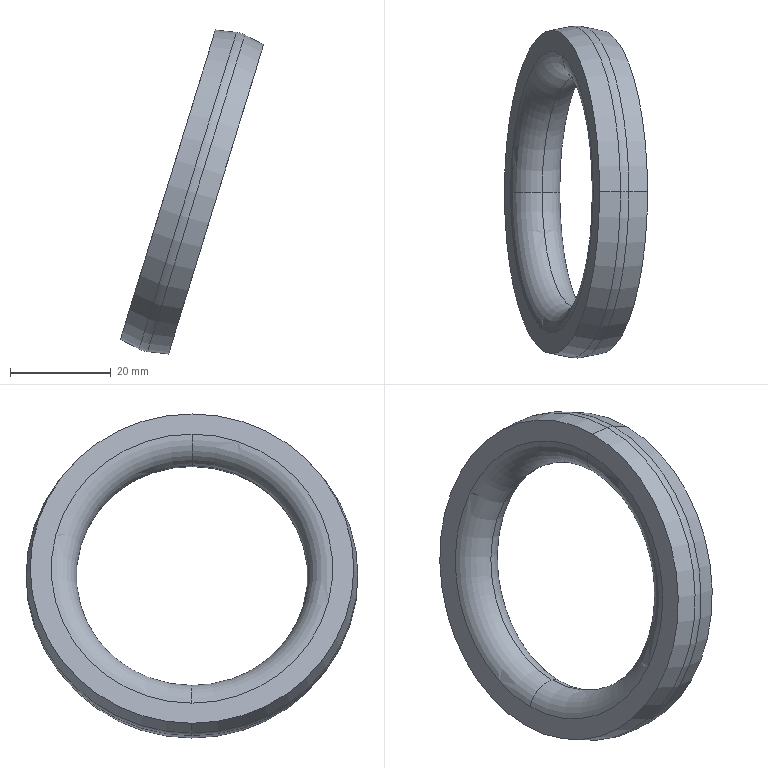Component | SolidWorks | DriveDevice-1_GuideWheelRubber-1 | 1 solid | 12 faces | box 28.47 x 66.09 x 64.5 mm | volume 15263 mm3 | torus 6 | cone 4 | plane 2
build123d program:
from build123d import *


with BuildPart() as part:
    # Sketch1 → Revolve1 (revolve)
    with BuildSketch(Plane(origin=(0, 0, 0), x_dir=(0, 0, -1), z_dir=(1, 0, 0)), mode=Mode.PRIVATE) as revolve1_sk:
        with BuildLine():
            Line((10, 28), (10, 32.2))
            Line((10, 32.2), (5.87, 32.964))
            ThreePointArc((5.87, 32.964), (5, 33.043), (4.13, 32.964))
            Line((4.13, 32.964), (0, 32.2))
            Line((0, 32.2), (0, 28))
            ThreePointArc((0, 28), (5, 23), (10, 28))
        make_face()
    revolve(revolve1_sk.sketch.rotate(Axis((0, 0, 5.5), (0, 0, -1)), 90), axis=Axis((0, 0, 5.5), (0, 0, -1)))


solid = part.part

# Placed as in the assembly
solid = solid.moved(Location((-210.893, 15, 15.882), (0, -72.922, -178.369)))
STEP:
#1=COLOUR_RGB('',0.7922,0.8196,0.9333);
#2=FILL_AREA_STYLE_COLOUR('',#1);
#3=FILL_AREA_STYLE('',(#2));
#4=SURFACE_STYLE_FILL_AREA(#3);
#5=SURFACE_SIDE_STYLE('',(#4));
#6=SURFACE_STYLE_USAGE(.BOTH.,#5);
#7=PRESENTATION_STYLE_ASSIGNMENT((#6));
#8=CARTESIAN_POINT('',(-8.381,0.5906,-0.2981));
#9=VERTEX_POINT('',#8);
#10=CARTESIAN_POINT('',(-8.25,0.5906,-0.5441));
#11=VERTEX_POINT('',#10);
#12=CARTESIAN_POINT('',(-8.438,0.5906,-0.4863));
#13=DIRECTION('',(-0.,1.,0.));
#14=DIRECTION('',(0.,-0.,1.));
#15=AXIS2_PLACEMENT_3D('',#12,#13,#14);
#16=CIRCLE('',#15,0.1969);
#17=EDGE_CURVE('',#9,#11,#16,.T.);
#18=ORIENTED_EDGE('',*,*,#17,.F.);
#19=CARTESIAN_POINT('',(-7.849,0.5906,1.433));
#20=VERTEX_POINT('',#19);
#21=CARTESIAN_POINT('',(-8.115,0.5906,0.5675));
#22=DIRECTION('',(-0.9559,-0.,0.2937));
#23=DIRECTION('',(0.2937,0.,0.9559));
#24=AXIS2_PLACEMENT_3D('',#21,#22,#23);
#25=CIRCLE('',#24,0.9055);
#26=EDGE_CURVE('',#9,#20,#25,.T.);
#27=ORIENTED_EDGE('',*,*,#26,.T.);
#28=CARTESIAN_POINT('',(-7.603,0.5906,1.563));
#29=VERTEX_POINT('',#28);
#30=CARTESIAN_POINT('',(-7.791,0.5906,1.621));
#31=DIRECTION('',(0.,-1.,-0.));
#32=DIRECTION('',(0.,0.,-1.));
#33=AXIS2_PLACEMENT_3D('',#30,#31,#32);
#34=CIRCLE('',#33,0.1969);
#35=EDGE_CURVE('',#20,#29,#34,.T.);
#36=ORIENTED_EDGE('',*,*,#35,.T.);
#37=CARTESIAN_POINT('',(-7.927,0.5906,0.5097));
#38=DIRECTION('',(-0.9559,-0.,0.2937));
#39=DIRECTION('',(0.2937,-0.,0.9559));
#40=AXIS2_PLACEMENT_3D('',#37,#38,#39);
#41=CIRCLE('',#40,1.102);
#42=EDGE_CURVE('',#11,#29,#41,.T.);
#43=ORIENTED_EDGE('',*,*,#42,.F.);
#44=EDGE_LOOP('',(#18,#27,#36,#43));
#45=FACE_OUTER_BOUND('',#44,.T.);
#46=CARTESIAN_POINT('',(-8.115,0.5906,0.5675));
#47=DIRECTION('',(-0.9559,-0.,0.2937));
#48=DIRECTION('',(0.2937,-0.,0.9559));
#49=AXIS2_PLACEMENT_3D('',#46,#47,#48);
#50=TOROIDAL_SURFACE('',#49,1.102,0.1969);
#51=ADVANCED_FACE('',(#45),#50,.T.);
#52=ORIENTED_EDGE('',*,*,#35,.F.);
#53=CARTESIAN_POINT('',(-8.115,0.5906,0.5675));
#54=DIRECTION('',(-0.9559,-0.,0.2937));
#55=DIRECTION('',(0.2937,0.,0.9559));
#56=AXIS2_PLACEMENT_3D('',#53,#54,#55);
#57=CIRCLE('',#56,0.9055);
#58=EDGE_CURVE('',#20,#9,#57,.T.);
#59=ORIENTED_EDGE('',*,*,#58,.T.);
#60=ORIENTED_EDGE('',*,*,#17,.T.);
#61=CARTESIAN_POINT('',(-7.927,0.5906,0.5097));
#62=DIRECTION('',(-0.9559,-0.,0.2937));
#63=DIRECTION('',(0.2937,-0.,0.9559));
#64=AXIS2_PLACEMENT_3D('',#61,#62,#63);
#65=CIRCLE('',#64,1.102);
#66=EDGE_CURVE('',#29,#11,#65,.T.);
#67=ORIENTED_EDGE('',*,*,#66,.F.);
#68=EDGE_LOOP('',(#52,#59,#60,#67));
#69=FACE_OUTER_BOUND('',#68,.T.);
#70=CARTESIAN_POINT('',(-8.115,0.5906,0.5675));
#71=DIRECTION('',(-0.9559,-0.,0.2937));
#72=DIRECTION('',(0.2937,-0.,0.9559));
#73=AXIS2_PLACEMENT_3D('',#70,#71,#72);
#74=TOROIDAL_SURFACE('',#73,1.102,0.1969);
#75=ADVANCED_FACE('',(#69),#74,.T.);
#76=CARTESIAN_POINT('',(-7.931,0.5906,1.837));
#77=VERTEX_POINT('',#76);
#78=CARTESIAN_POINT('',(-8.675,0.5906,-0.5865));
#79=VERTEX_POINT('',#78);
#80=CARTESIAN_POINT('',(-8.303,0.5906,0.6253));
#81=DIRECTION('',(-0.9559,-0.,0.2937));
#82=DIRECTION('',(0.2937,-0.,0.9559));
#83=AXIS2_PLACEMENT_3D('',#80,#81,#82);
#84=CIRCLE('',#83,1.268);
#85=EDGE_CURVE('',#77,#79,#84,.T.);
#86=ORIENTED_EDGE('',*,*,#85,.F.);
#87=CARTESIAN_POINT('',(-7.766,0.5906,1.818));
#88=VERTEX_POINT('',#87);
#89=CARTESIAN_POINT('',(-7.766,0.5906,1.818));
#90=DIRECTION('',(0.9934,0.,-0.115));
#91=VECTOR('',#90,39.37);
#92=LINE('',#89,#91);
#93=EDGE_CURVE('',#77,#88,#92,.T.);
#94=ORIENTED_EDGE('',*,*,#93,.T.);
#95=CARTESIAN_POINT('',(-8.529,0.5906,-0.663));
#96=VERTEX_POINT('',#95);
#97=CARTESIAN_POINT('',(-8.147,0.5906,0.5775));
#98=DIRECTION('',(-0.9559,-0.,0.2937));
#99=DIRECTION('',(0.2937,-0.,0.9559));
#100=AXIS2_PLACEMENT_3D('',#97,#98,#99);
#101=CIRCLE('',#100,1.298);
#102=EDGE_CURVE('',#88,#96,#101,.T.);
#103=ORIENTED_EDGE('',*,*,#102,.T.);
#104=CARTESIAN_POINT('',(-8.529,0.5906,-0.663));
#105=DIRECTION('',(0.8866,0.,-0.4626));
#106=VECTOR('',#105,39.37);
#107=LINE('',#104,#106);
#108=EDGE_CURVE('',#79,#96,#107,.T.);
#109=ORIENTED_EDGE('',*,*,#108,.F.);
#110=EDGE_LOOP('',(#86,#94,#103,#109));
#111=FACE_OUTER_BOUND('',#110,.T.);
#112=CARTESIAN_POINT('',(-8.147,0.5906,0.5775));
#113=DIRECTION('',(0.9559,0.,-0.2937));
#114=DIRECTION('',(-0.2937,0.,-0.9559));
#115=AXIS2_PLACEMENT_3D('',#112,#113,#114);
#116=CONICAL_SURFACE('',#115,1.298,0.1828);
#117=ADVANCED_FACE('',(#111),#116,.T.);
#118=CARTESIAN_POINT('',(-7.701,0.5906,1.798));
#119=VERTEX_POINT('',#118);
#120=CARTESIAN_POINT('',(-8.463,0.5906,-0.6831));
#121=VERTEX_POINT('',#120);
#122=CARTESIAN_POINT('',(-8.082,0.5906,0.5574));
#123=DIRECTION('',(-0.9559,-0.,0.2937));
#124=DIRECTION('',(0.2937,-0.,0.9559));
#125=AXIS2_PLACEMENT_3D('',#122,#123,#124);
#126=CIRCLE('',#125,1.298);
#127=EDGE_CURVE('',#119,#121,#126,.T.);
#128=ORIENTED_EDGE('',*,*,#127,.T.);
#129=CARTESIAN_POINT('',(-8.441,0.5906,-0.496));
#130=DIRECTION('',(-0.,1.,0.));
#131=DIRECTION('',(0.,-0.,1.));
#132=AXIS2_PLACEMENT_3D('',#129,#130,#131);
#133=CIRCLE('',#132,0.1884);
#134=EDGE_CURVE('',#121,#96,#133,.T.);
#135=ORIENTED_EDGE('',*,*,#134,.T.);
#136=ORIENTED_EDGE('',*,*,#102,.F.);
#137=CARTESIAN_POINT('',(-7.788,0.5906,1.631));
#138=DIRECTION('',(0.,-1.,-0.));
#139=DIRECTION('',(0.,0.,-1.));
#140=AXIS2_PLACEMENT_3D('',#137,#138,#139);
#141=CIRCLE('',#140,0.1884);
#142=EDGE_CURVE('',#119,#88,#141,.T.);
#143=ORIENTED_EDGE('',*,*,#142,.F.);
#144=EDGE_LOOP('',(#128,#135,#136,#143));
#145=FACE_OUTER_BOUND('',#144,.T.);
#146=CARTESIAN_POINT('',(-8.115,0.5906,0.5675));
#147=DIRECTION('',(-0.9559,-0.,0.2937));
#148=DIRECTION('',(0.2937,-0.,0.9559));
#149=AXIS2_PLACEMENT_3D('',#146,#147,#148);
#150=TOROIDAL_SURFACE('',#149,1.113,0.1884);
#151=ADVANCED_FACE('',(#145),#150,.T.);
#152=CARTESIAN_POINT('',(-7.554,0.5906,1.721));
#153=VERTEX_POINT('',#152);
#154=CARTESIAN_POINT('',(-8.299,0.5906,-0.7022));
#155=VERTEX_POINT('',#154);
#156=CARTESIAN_POINT('',(-7.927,0.5906,0.5097));
#157=DIRECTION('',(-0.9559,-0.,0.2937));
#158=DIRECTION('',(0.2937,-0.,0.9559));
#159=AXIS2_PLACEMENT_3D('',#156,#157,#158);
#160=CIRCLE('',#159,1.268);
#161=EDGE_CURVE('',#153,#155,#160,.T.);
#162=ORIENTED_EDGE('',*,*,#161,.T.);
#163=CARTESIAN_POINT('',(-8.299,0.5906,-0.7022));
#164=DIRECTION('',(-0.9934,-0.,0.115));
#165=VECTOR('',#164,39.37);
#166=LINE('',#163,#165);
#167=EDGE_CURVE('',#155,#121,#166,.T.);
#168=ORIENTED_EDGE('',*,*,#167,.T.);
#169=ORIENTED_EDGE('',*,*,#127,.F.);
#170=CARTESIAN_POINT('',(-7.554,0.5906,1.721));
#171=DIRECTION('',(-0.8866,-0.,0.4626));
#172=VECTOR('',#171,39.37);
#173=LINE('',#170,#172);
#174=EDGE_CURVE('',#153,#119,#173,.T.);
#175=ORIENTED_EDGE('',*,*,#174,.F.);
#176=EDGE_LOOP('',(#162,#168,#169,#175));
#177=FACE_OUTER_BOUND('',#176,.T.);
#178=CARTESIAN_POINT('',(-7.927,0.5906,0.5097));
#179=DIRECTION('',(-0.9559,-0.,0.2937));
#180=DIRECTION('',(0.2937,-0.,0.9559));
#181=AXIS2_PLACEMENT_3D('',#178,#179,#180);
#182=CONICAL_SURFACE('',#181,1.268,0.1828);
#183=ADVANCED_FACE('',(#177),#182,.T.);
#184=ORIENTED_EDGE('',*,*,#58,.F.);
#185=CARTESIAN_POINT('',(-7.979,0.5906,1.679));
#186=VERTEX_POINT('',#185);
#187=CARTESIAN_POINT('',(-7.791,0.5906,1.621));
#188=DIRECTION('',(0.,-1.,-0.));
#189=DIRECTION('',(0.,0.,-1.));
#190=AXIS2_PLACEMENT_3D('',#187,#188,#189);
#191=CIRCLE('',#190,0.1969);
#192=EDGE_CURVE('',#186,#20,#191,.T.);
#193=ORIENTED_EDGE('',*,*,#192,.F.);
#194=CARTESIAN_POINT('',(-8.627,0.5906,-0.4285));
#195=VERTEX_POINT('',#194);
#196=CARTESIAN_POINT('',(-8.303,0.5906,0.6253));
#197=DIRECTION('',(-0.9559,-0.,0.2937));
#198=DIRECTION('',(0.2937,-0.,0.9559));
#199=AXIS2_PLACEMENT_3D('',#196,#197,#198);
#200=CIRCLE('',#199,1.102);
#201=EDGE_CURVE('',#186,#195,#200,.T.);
#202=ORIENTED_EDGE('',*,*,#201,.T.);
#203=CARTESIAN_POINT('',(-8.438,0.5906,-0.4863));
#204=DIRECTION('',(-0.,1.,0.));
#205=DIRECTION('',(0.,-0.,1.));
#206=AXIS2_PLACEMENT_3D('',#203,#204,#205);
#207=CIRCLE('',#206,0.1969);
#208=EDGE_CURVE('',#195,#9,#207,.T.);
#209=ORIENTED_EDGE('',*,*,#208,.T.);
#210=EDGE_LOOP('',(#184,#193,#202,#209));
#211=FACE_OUTER_BOUND('',#210,.T.);
#212=CARTESIAN_POINT('',(-8.115,0.5906,0.5675));
#213=DIRECTION('',(-0.9559,-0.,0.2937));
#214=DIRECTION('',(0.2937,-0.,0.9559));
#215=AXIS2_PLACEMENT_3D('',#212,#213,#214);
#216=TOROIDAL_SURFACE('',#215,1.102,0.1969);
#217=ADVANCED_FACE('',(#211),#216,.T.);
#218=ORIENTED_EDGE('',*,*,#26,.F.);
#219=ORIENTED_EDGE('',*,*,#208,.F.);
#220=CARTESIAN_POINT('',(-8.303,0.5906,0.6253));
#221=DIRECTION('',(-0.9559,-0.,0.2937));
#222=DIRECTION('',(0.2937,-0.,0.9559));
#223=AXIS2_PLACEMENT_3D('',#220,#221,#222);
#224=CIRCLE('',#223,1.102);
#225=EDGE_CURVE('',#195,#186,#224,.T.);
#226=ORIENTED_EDGE('',*,*,#225,.T.);
#227=ORIENTED_EDGE('',*,*,#192,.T.);
#228=EDGE_LOOP('',(#218,#219,#226,#227));
#229=FACE_OUTER_BOUND('',#228,.T.);
#230=CARTESIAN_POINT('',(-8.115,0.5906,0.5675));
#231=DIRECTION('',(-0.9559,-0.,0.2937));
#232=DIRECTION('',(0.2937,-0.,0.9559));
#233=AXIS2_PLACEMENT_3D('',#230,#231,#232);
#234=TOROIDAL_SURFACE('',#233,1.102,0.1969);
#235=ADVANCED_FACE('',(#229),#234,.T.);
#236=ORIENTED_EDGE('',*,*,#161,.F.);
#237=CARTESIAN_POINT('',(-7.927,0.5906,0.5097));
#238=DIRECTION('',(-0.9559,-0.,0.2937));
#239=DIRECTION('',(0.2937,-0.,0.9559));
#240=AXIS2_PLACEMENT_3D('',#237,#238,#239);
#241=CIRCLE('',#240,1.268);
#242=EDGE_CURVE('',#155,#153,#241,.T.);
#243=ORIENTED_EDGE('',*,*,#242,.F.);
#244=EDGE_LOOP('',(#236,#243));
#245=FACE_OUTER_BOUND('',#244,.T.);
#246=ORIENTED_EDGE('',*,*,#66,.T.);
#247=ORIENTED_EDGE('',*,*,#42,.T.);
#248=EDGE_LOOP('',(#246,#247));
#249=FACE_BOUND('',#248,.T.);
#250=CARTESIAN_POINT('',(-7.927,1.693,0.5097));
#251=DIRECTION('',(-0.9559,-0.,0.2937));
#252=DIRECTION('',(0.2937,-0.,0.9559));
#253=AXIS2_PLACEMENT_3D('',#250,#251,#252);
#254=PLANE('',#253);
#255=ADVANCED_FACE('',(#245,#249),#254,.F.);
#256=ORIENTED_EDGE('',*,*,#167,.F.);
#257=ORIENTED_EDGE('',*,*,#242,.T.);
#258=ORIENTED_EDGE('',*,*,#174,.T.);
#259=CARTESIAN_POINT('',(-8.082,0.5906,0.5574));
#260=DIRECTION('',(-0.9559,-0.,0.2937));
#261=DIRECTION('',(0.2937,-0.,0.9559));
#262=AXIS2_PLACEMENT_3D('',#259,#260,#261);
#263=CIRCLE('',#262,1.298);
#264=EDGE_CURVE('',#121,#119,#263,.T.);
#265=ORIENTED_EDGE('',*,*,#264,.F.);
#266=EDGE_LOOP('',(#256,#257,#258,#265));
#267=FACE_OUTER_BOUND('',#266,.T.);
#268=CARTESIAN_POINT('',(-7.927,0.5906,0.5097));
#269=DIRECTION('',(-0.9559,-0.,0.2937));
#270=DIRECTION('',(0.2937,-0.,0.9559));
#271=AXIS2_PLACEMENT_3D('',#268,#269,#270);
#272=CONICAL_SURFACE('',#271,1.268,0.1828);
#273=ADVANCED_FACE('',(#267),#272,.T.);
#274=ORIENTED_EDGE('',*,*,#134,.F.);
#275=ORIENTED_EDGE('',*,*,#264,.T.);
#276=ORIENTED_EDGE('',*,*,#142,.T.);
#277=CARTESIAN_POINT('',(-8.147,0.5906,0.5775));
#278=DIRECTION('',(-0.9559,-0.,0.2937));
#279=DIRECTION('',(0.2937,-0.,0.9559));
#280=AXIS2_PLACEMENT_3D('',#277,#278,#279);
#281=CIRCLE('',#280,1.298);
#282=EDGE_CURVE('',#96,#88,#281,.T.);
#283=ORIENTED_EDGE('',*,*,#282,.F.);
#284=EDGE_LOOP('',(#274,#275,#276,#283));
#285=FACE_OUTER_BOUND('',#284,.T.);
#286=CARTESIAN_POINT('',(-8.115,0.5906,0.5675));
#287=DIRECTION('',(-0.9559,-0.,0.2937));
#288=DIRECTION('',(0.2937,-0.,0.9559));
#289=AXIS2_PLACEMENT_3D('',#286,#287,#288);
#290=TOROIDAL_SURFACE('',#289,1.113,0.1884);
#291=ADVANCED_FACE('',(#285),#290,.T.);
#292=ORIENTED_EDGE('',*,*,#93,.F.);
#293=CARTESIAN_POINT('',(-8.303,0.5906,0.6253));
#294=DIRECTION('',(-0.9559,-0.,0.2937));
#295=DIRECTION('',(0.2937,-0.,0.9559));
#296=AXIS2_PLACEMENT_3D('',#293,#294,#295);
#297=CIRCLE('',#296,1.268);
#298=EDGE_CURVE('',#79,#77,#297,.T.);
#299=ORIENTED_EDGE('',*,*,#298,.F.);
#300=ORIENTED_EDGE('',*,*,#108,.T.);
#301=ORIENTED_EDGE('',*,*,#282,.T.);
#302=EDGE_LOOP('',(#292,#299,#300,#301));
#303=FACE_OUTER_BOUND('',#302,.T.);
#304=CARTESIAN_POINT('',(-8.147,0.5906,0.5775));
#305=DIRECTION('',(0.9559,0.,-0.2937));
#306=DIRECTION('',(-0.2937,0.,-0.9559));
#307=AXIS2_PLACEMENT_3D('',#304,#305,#306);
#308=CONICAL_SURFACE('',#307,1.298,0.1828);
#309=ADVANCED_FACE('',(#303),#308,.T.);
#310=ORIENTED_EDGE('',*,*,#201,.F.);
#311=ORIENTED_EDGE('',*,*,#225,.F.);
#312=EDGE_LOOP('',(#310,#311));
#313=FACE_BOUND('',#312,.T.);
#314=ORIENTED_EDGE('',*,*,#298,.T.);
#315=ORIENTED_EDGE('',*,*,#85,.T.);
#316=EDGE_LOOP('',(#314,#315));
#317=FACE_OUTER_BOUND('',#316,.T.);
#318=CARTESIAN_POINT('',(-8.303,1.858,0.6253));
#319=DIRECTION('',(0.9559,0.,-0.2937));
#320=DIRECTION('',(-0.2937,0.,-0.9559));
#321=AXIS2_PLACEMENT_3D('',#318,#319,#320);
#322=PLANE('',#321);
#323=ADVANCED_FACE('',(#313,#317),#322,.F.);
#324=CLOSED_SHELL('',(#51,#75,#117,#151,#183,#217,#235,#255,#273,#291,#309,#323));
#325=MANIFOLD_SOLID_BREP('',#324);
#326=STYLED_ITEM('',(#7),#325);
#327=(LENGTH_UNIT()NAMED_UNIT(*)SI_UNIT($,.METRE.));
#328=LENGTH_MEASURE_WITH_UNIT(LENGTH_MEASURE(0.0254),#327);
#329=DIMENSIONAL_EXPONENTS(1.,0.,0.,0.,0.,0.,0.);
#330=(CONVERSION_BASED_UNIT('',#328)LENGTH_UNIT()NAMED_UNIT(#329));
#331=UNCERTAINTY_MEASURE_WITH_UNIT(LENGTH_MEASURE(0.00001),#330,'','');
#332=(NAMED_UNIT(*)PLANE_ANGLE_UNIT()SI_UNIT($,.RADIAN.));
#333=(NAMED_UNIT(*)SI_UNIT($,.STERADIAN.)SOLID_ANGLE_UNIT());
#334=(GEOMETRIC_REPRESENTATION_CONTEXT(3)GLOBAL_UNCERTAINTY_ASSIGNED_CONTEXT((#331))GLOBAL_UNIT_ASSIGNED_CONTEXT((#330,#332,#333))REPRESENTATION_CONTEXT('',''));
#335=MECHANICAL_DESIGN_GEOMETRIC_PRESENTATION_REPRESENTATION('',(#326),#334);
#336=PRESENTATION_LAYER_ASSIGNMENT('','',(#326));
#337=CARTESIAN_POINT('',(0.,0.,0.));
#338=DIRECTION('',(0.,0.,1.));
#339=DIRECTION('',(1.,0.,0.));
#340=AXIS2_PLACEMENT_3D('',#337,#338,#339);
#341=(LENGTH_UNIT()NAMED_UNIT(*)SI_UNIT($,.METRE.));
#342=LENGTH_MEASURE_WITH_UNIT(LENGTH_MEASURE(0.0254),#341);
#343=DIMENSIONAL_EXPONENTS(1.,0.,0.,0.,0.,0.,0.);
#344=(CONVERSION_BASED_UNIT('',#342)LENGTH_UNIT()NAMED_UNIT(#343));
#345=UNCERTAINTY_MEASURE_WITH_UNIT(LENGTH_MEASURE(0.00001),#344,'','');
#346=(NAMED_UNIT(*)PLANE_ANGLE_UNIT()SI_UNIT($,.RADIAN.));
#347=(NAMED_UNIT(*)SI_UNIT($,.STERADIAN.)SOLID_ANGLE_UNIT());
#348=(GEOMETRIC_REPRESENTATION_CONTEXT(3)GLOBAL_UNCERTAINTY_ASSIGNED_CONTEXT((#345))GLOBAL_UNIT_ASSIGNED_CONTEXT((#344,#346,#347))REPRESENTATION_CONTEXT('',''));
#349=ADVANCED_BREP_SHAPE_REPRESENTATION('',(#325,#340),#348);